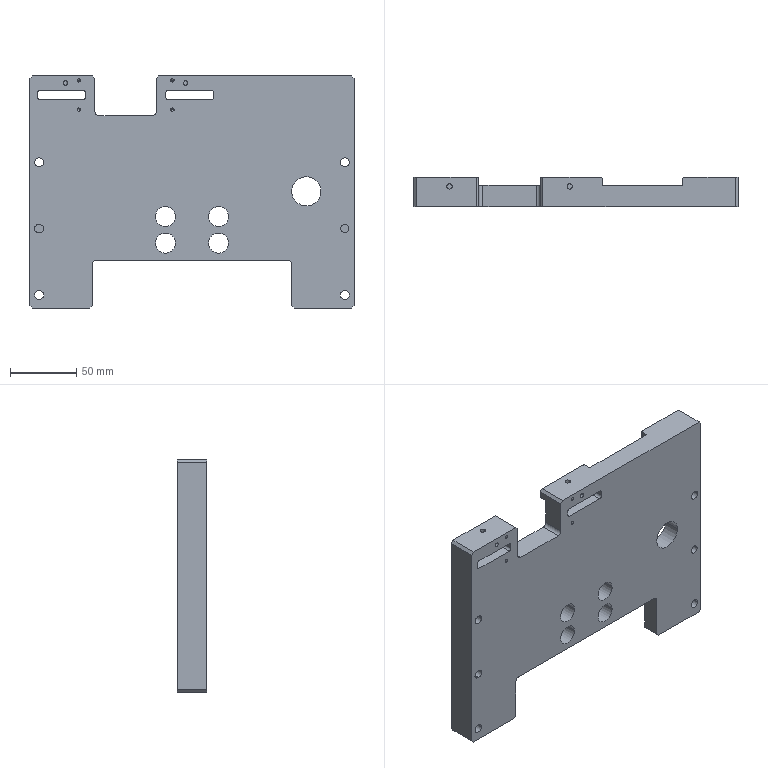Component | SolidWorks | SAWH02-03102A0MountingPlate2-1 | 1 solid | 196 faces | box 244 x 22 x 175 mm | volume 523550 mm3 | cylinder 108 | plane 68 | cone 8 | spline 8 | torus 4 | commonest cylinder face diameters 3 x24 4 x16 2 x15 6 x12 15 x8 2.5 x8 11 x8 6.6 x8 | material Light Green Fiberglass Board